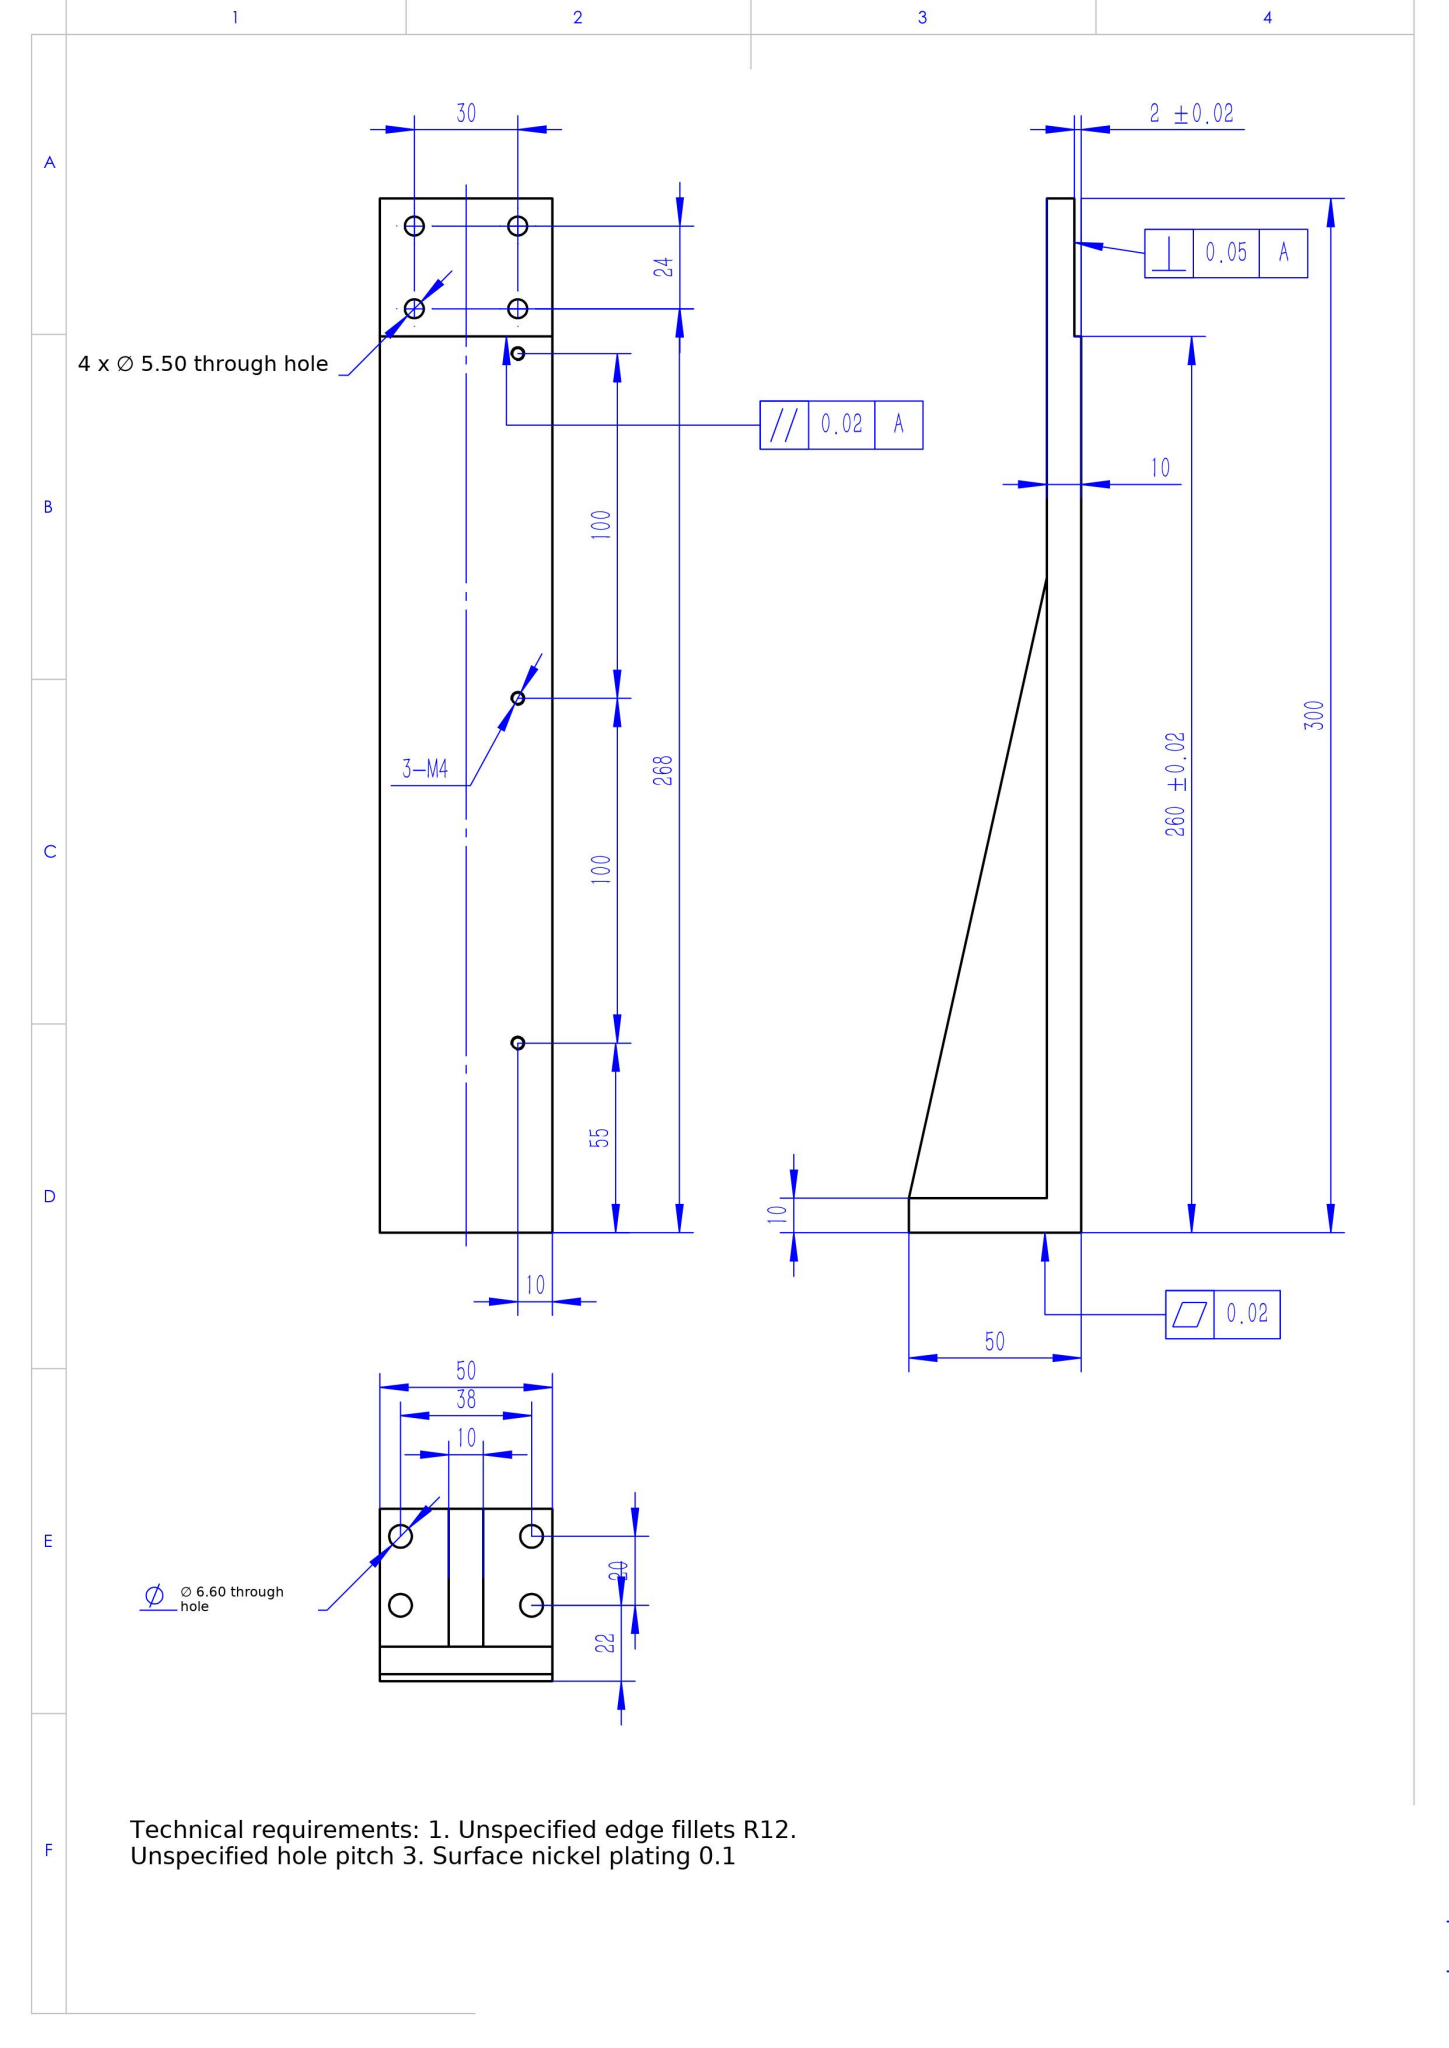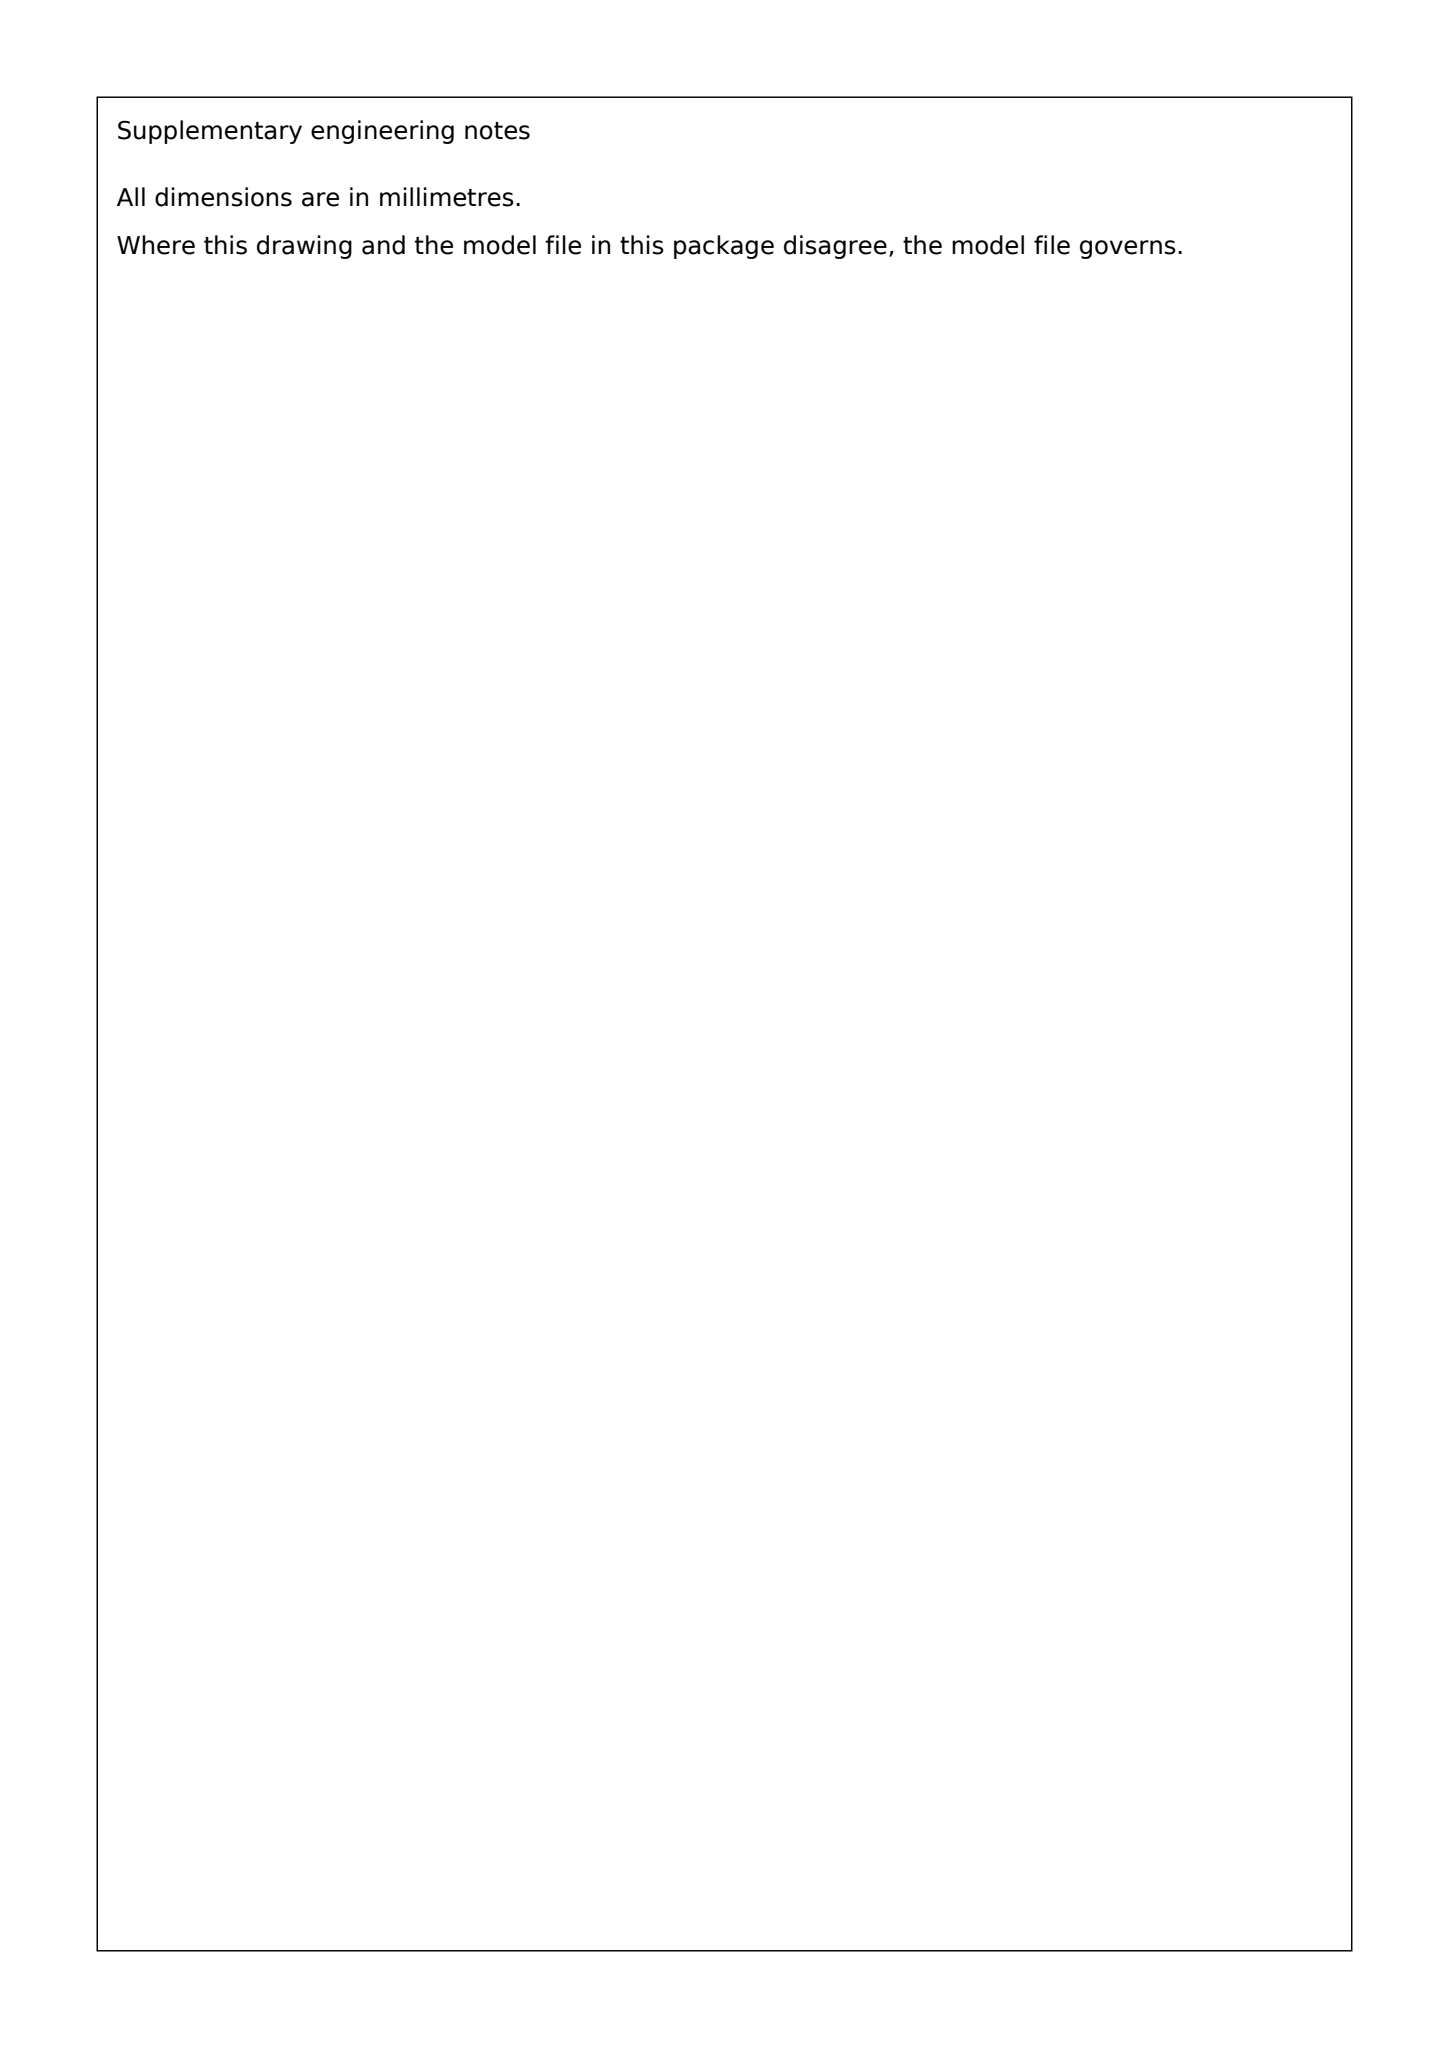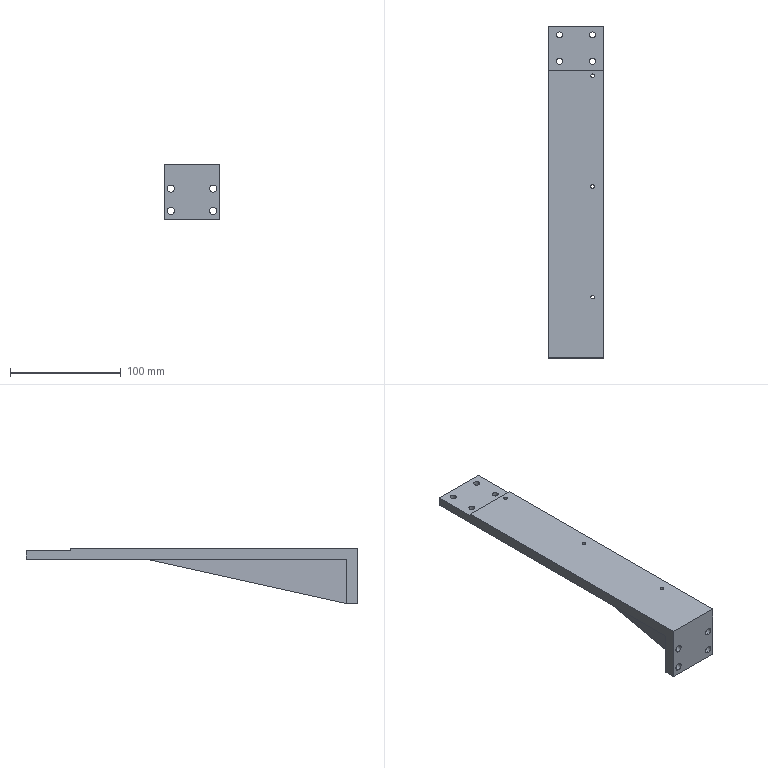Part | SolidWorks | mm | 1 solid | 36 faces | box 50 x 300 x 50 mm | volume 197979 mm3 | cylinder 22 | plane 14 | commonest cylinder face diameters 5.5 x8 6.6 x8 3.3 x6
build123d program:
from build123d import *

# Parameters (mm, degrees)
BOSS_EXTRUDE1_DEPTH  = 25
RIB1_REACH           = 307.164
SKETCH3_WALL_W       = 796.719
SKETCH3_WALL_H       = 10
RIB1_DRAFT_ANGLE     = -1
M6_CLEARANCE_HOLE1_D = 6.6
SKETCH6_W            = 50
SKETCH6_H            = 40
CUT_EXTRUDE1_DEPTH   = 2
M5_CLEARANCE_HOLE1_D = 5.5
M4_TAPPED_HOLE1_D    = 3.3
LPATTERN1_COUNT      = 3
LPATTERN1_PITCH      = 100


with BuildPart() as part:
    # Sketch1 → Boss-Extrude1 (new, symmetric)
    with BuildSketch(Plane(origin=(0, 0, 0), x_dir=(0, 0, -1), z_dir=(1, 0, 0))):
        Polygon((0, 0), (50, 0), (50, 10), (10, 10), (10, 300), (0, 300), align=None)
    extrude(amount=BOSS_EXTRUDE1_DEPTH, both=True)

    # Sketch3 wall → Rib1 (add, up to next)
    with BuildSketch(Plane(origin=(0, 100, -30), x_dir=(0, 0.9762, 0.2169), z_dir=(0, -0.2169, 0.9762)), mode=Mode.PRIVATE) as rib1_sk1:
        Rectangle(SKETCH3_WALL_W, SKETCH3_WALL_H)
    rib1_tool1 = extrude(rib1_sk1.sketch, amount=RIB1_REACH, mode=Mode.PRIVATE) - part.part
    add(rib1_tool1.solids().sort_by_distance((0, 100, -30))[0])

    # Rib1 draft
    rib1_draft_faces = [part.faces().sort_by_distance(p)[0] for p in [
        (-5, 99.892, -29.512),
        (5, 99.892, -29.512),
    ]]
    draft(rib1_draft_faces, Plane(origin=(0, 100, -30), x_dir=(0, 0.9762, 0.2169), z_dir=(0, 0.2169, -0.9762)), RIB1_DRAFT_ANGLE)

    # M6 Clearance Hole1 (through all)
    with Locations(Plane(origin=(0, 10, 0), x_dir=(1, 0, 0), z_dir=(0, 1, 0))):
        with Locations((-19, 42), (-19, 22), (19, 22), (19, 42)):
            Hole(M6_CLEARANCE_HOLE1_D / 2)

    # Sketch6 → Cut-Extrude1 (cut)
    with BuildSketch(Plane.XY):
        with Locations((0, 280)):
            Rectangle(SKETCH6_W, SKETCH6_H)
    extrude(amount=-CUT_EXTRUDE1_DEPTH, mode=Mode.SUBTRACT)

    # M5 Clearance Hole1 (through all)
    with Locations(Plane.XY.offset(-2)):
        with Locations((-15, 292), (15, 268), (15, 292), (-15, 268)):
            Hole(M5_CLEARANCE_HOLE1_D / 2)

    # M4 Tapped Hole1 (through all)
    with Locations(Plane(origin=(0, 0, -10), x_dir=(-1, 0, 0), z_dir=(0, 0, -1))):
        with Locations((-15, 255)):
            m4_tapped_hole1 = Hole(M4_TAPPED_HOLE1_D / 2)

    # LPattern1: M4 Tapped Hole1 ×3
    with Locations(*[(0, -i * LPATTERN1_PITCH, 0) for i in range(1, LPATTERN1_COUNT)]):
        add(m4_tapped_hole1, mode=Mode.SUBTRACT)


solid = part.part